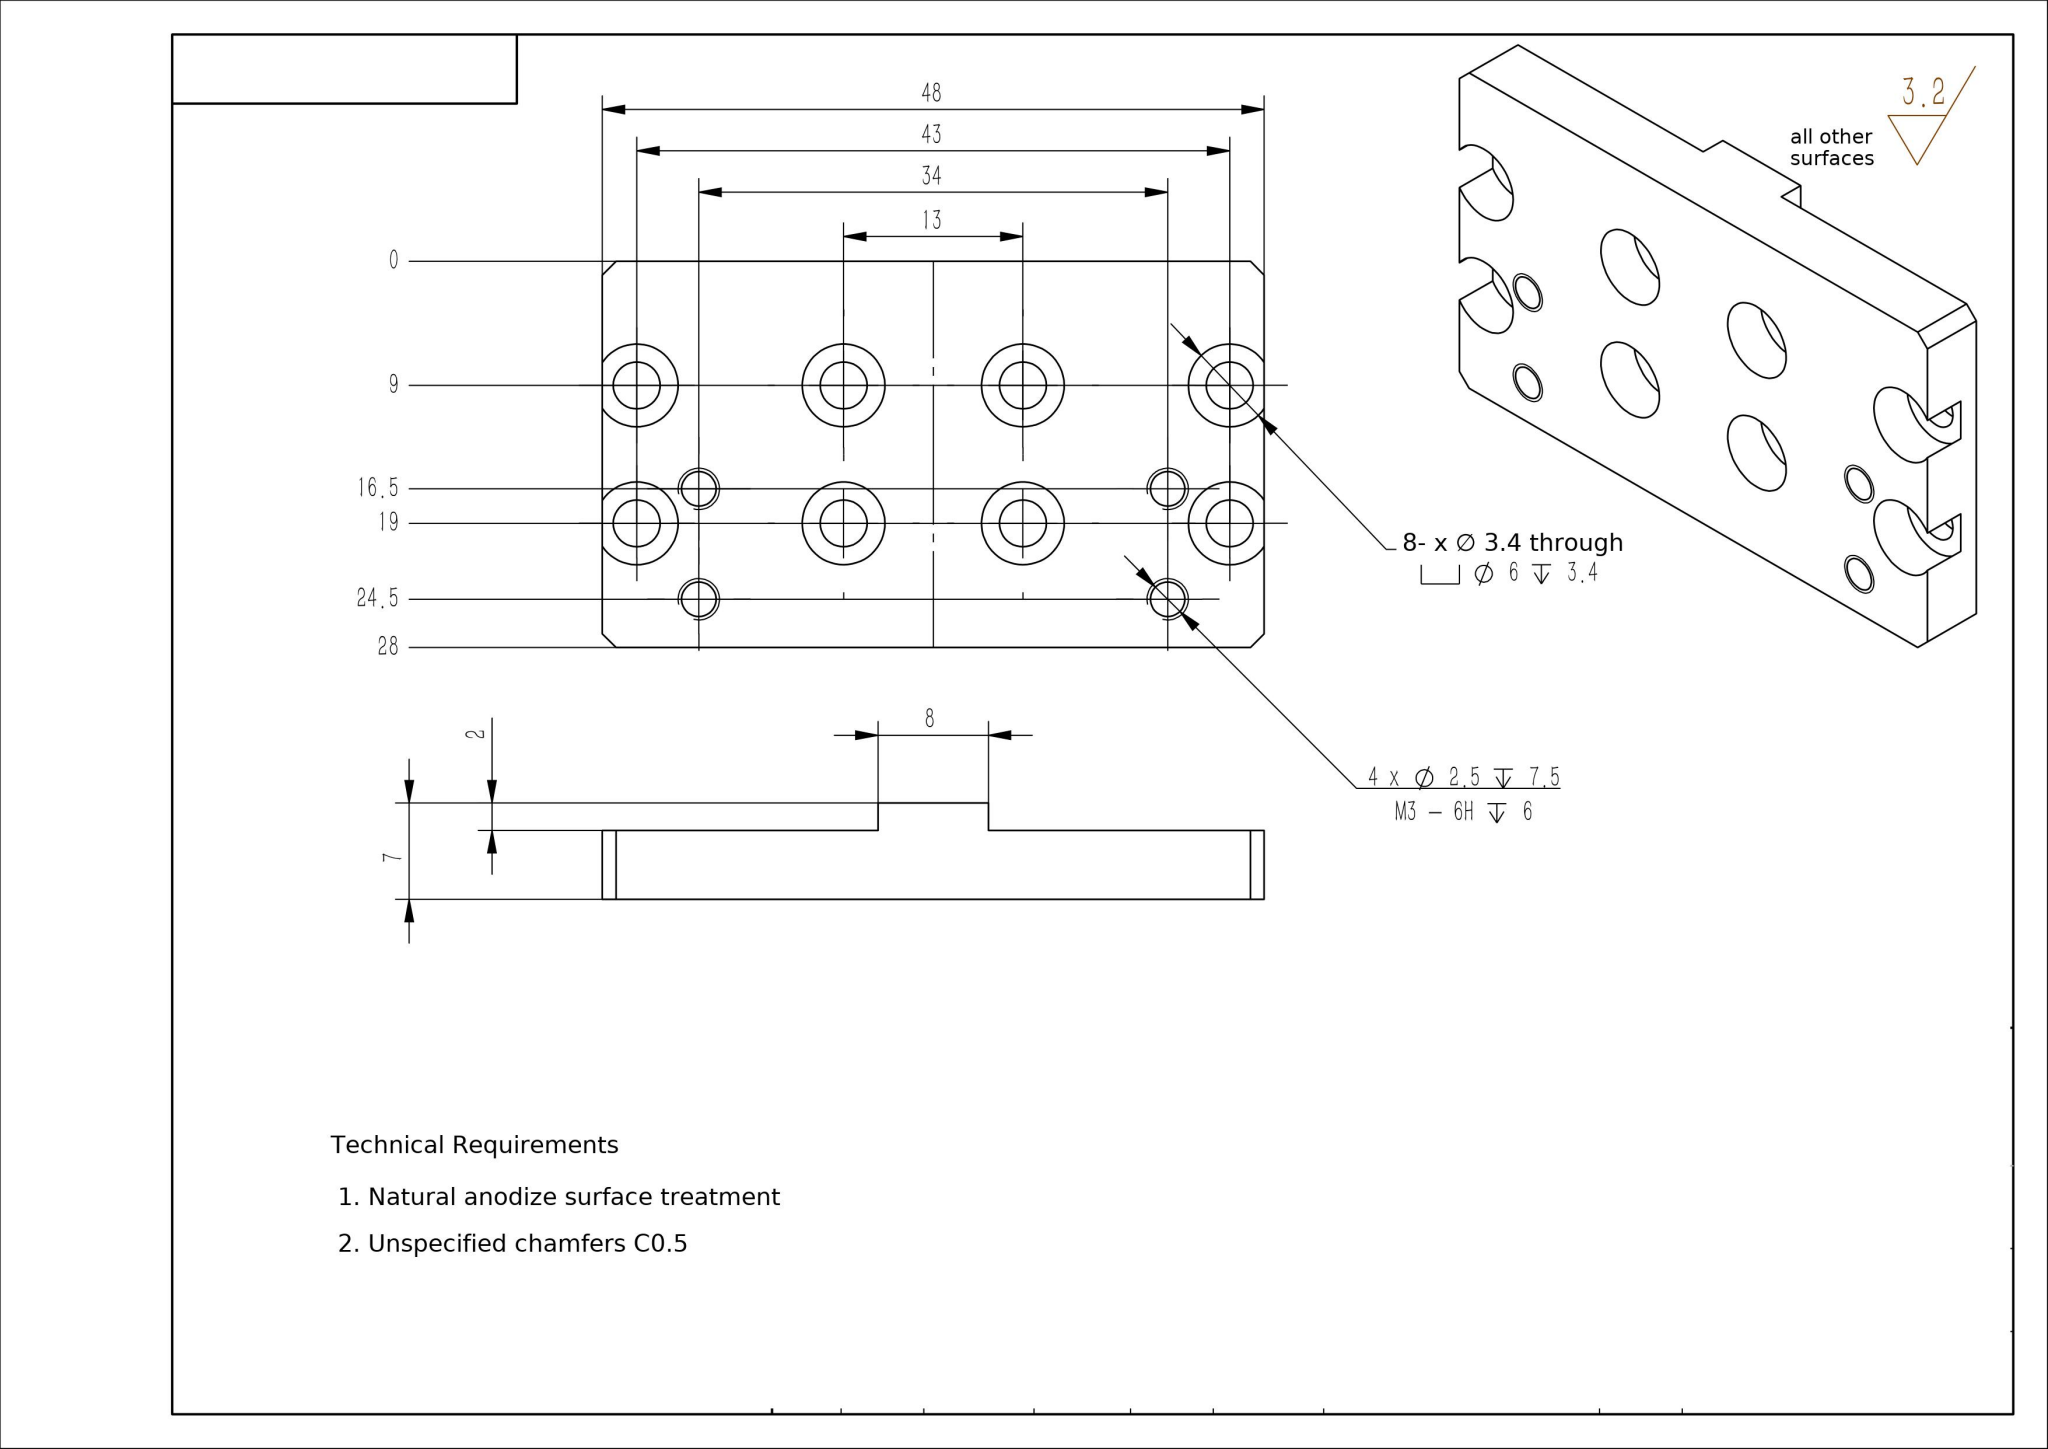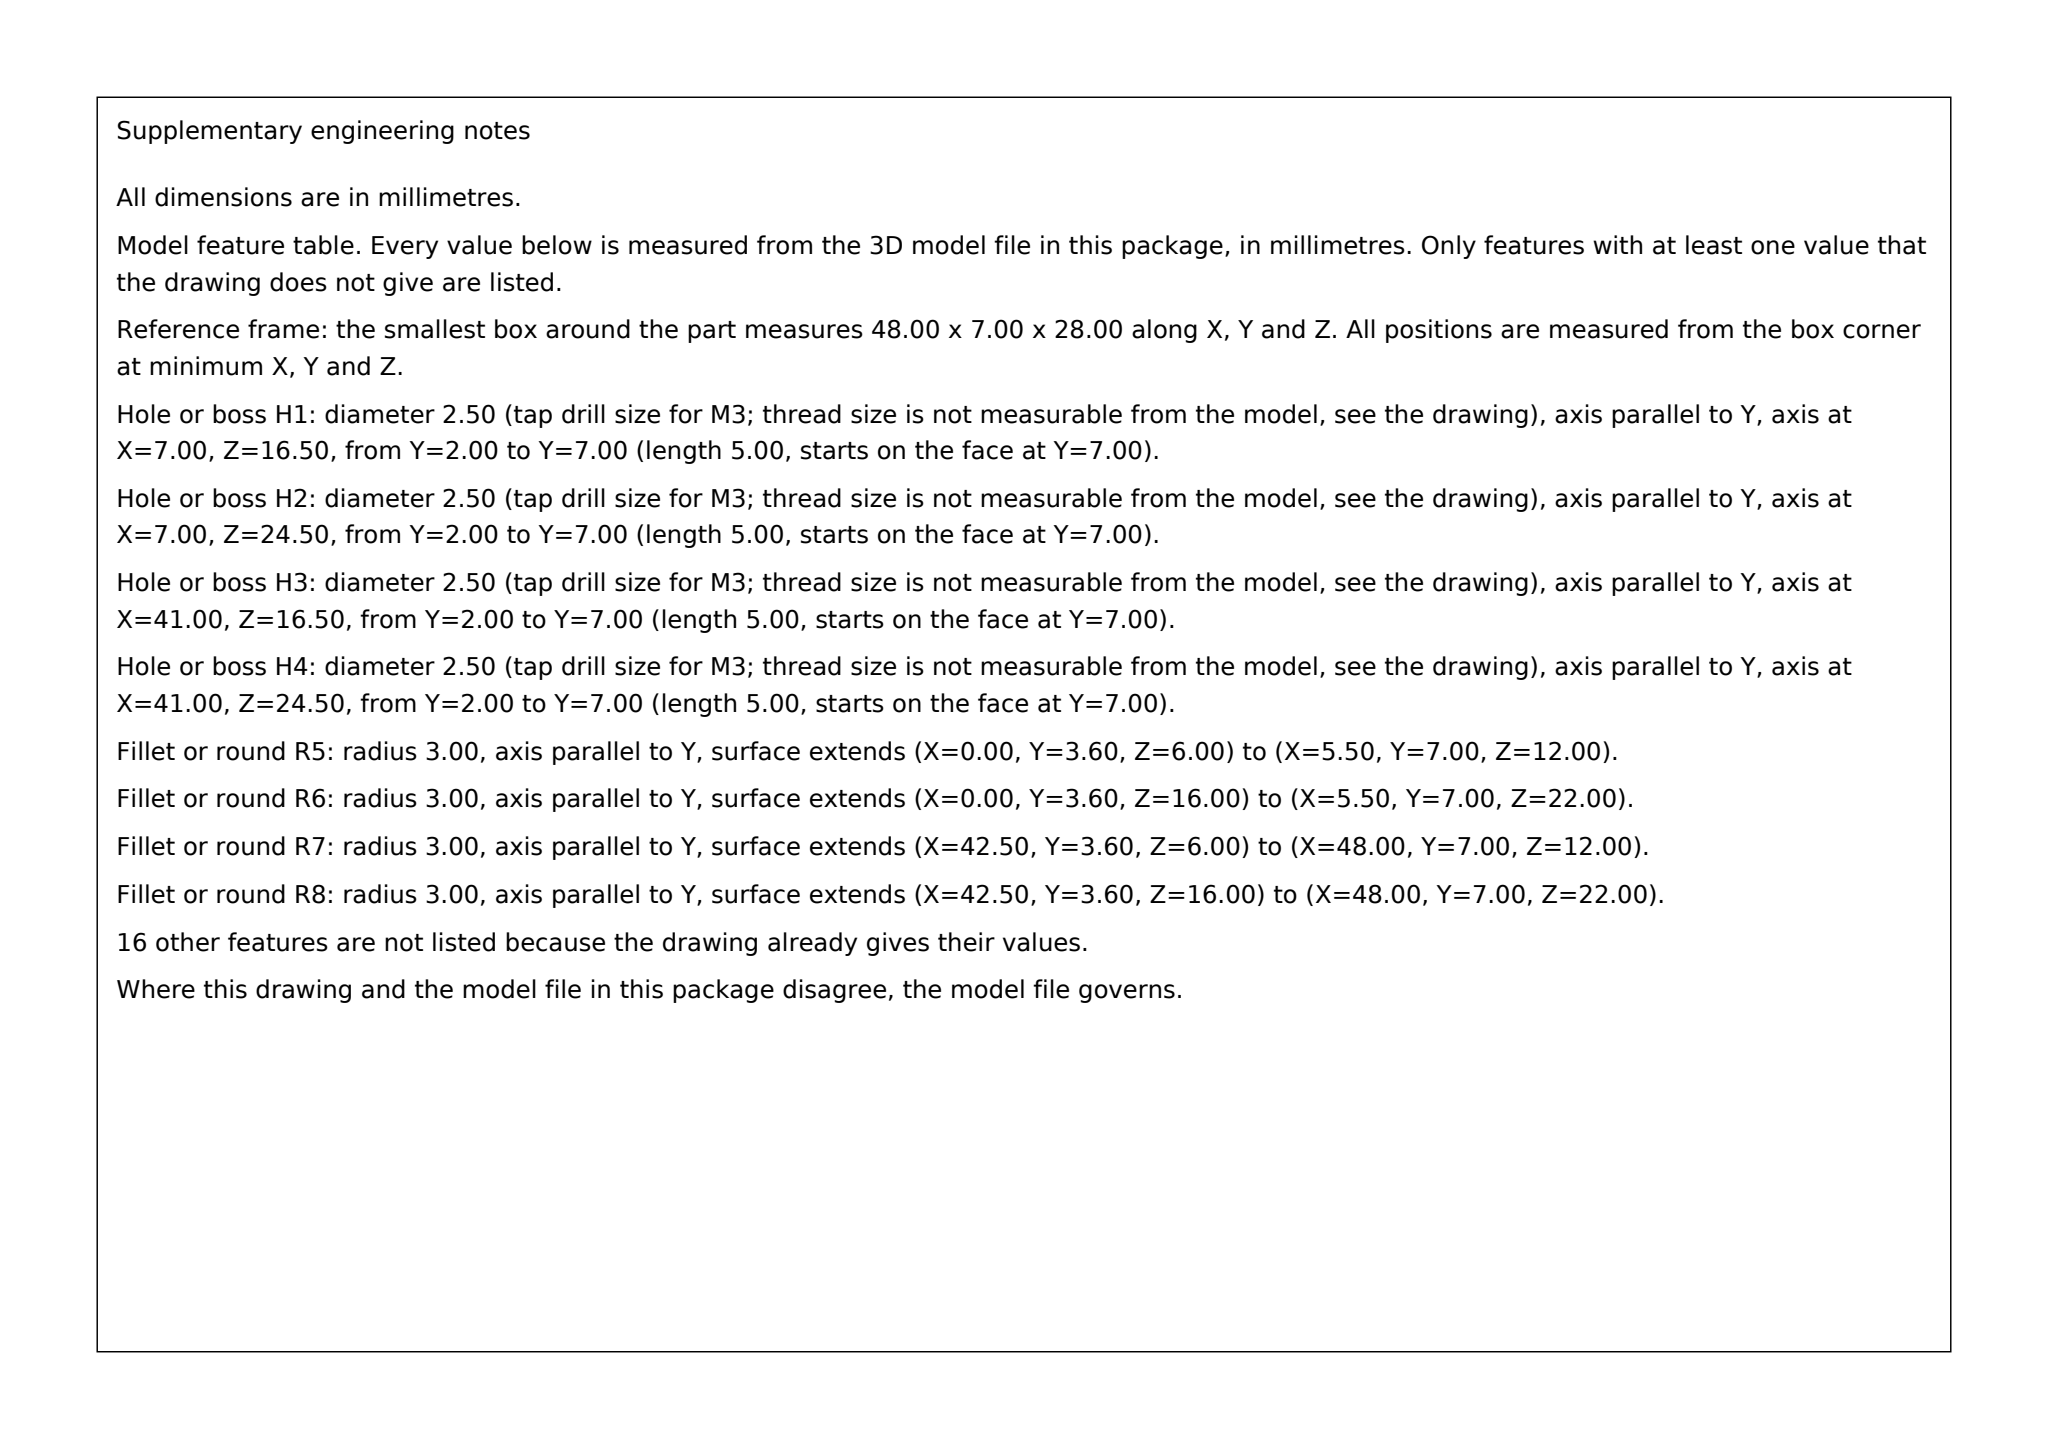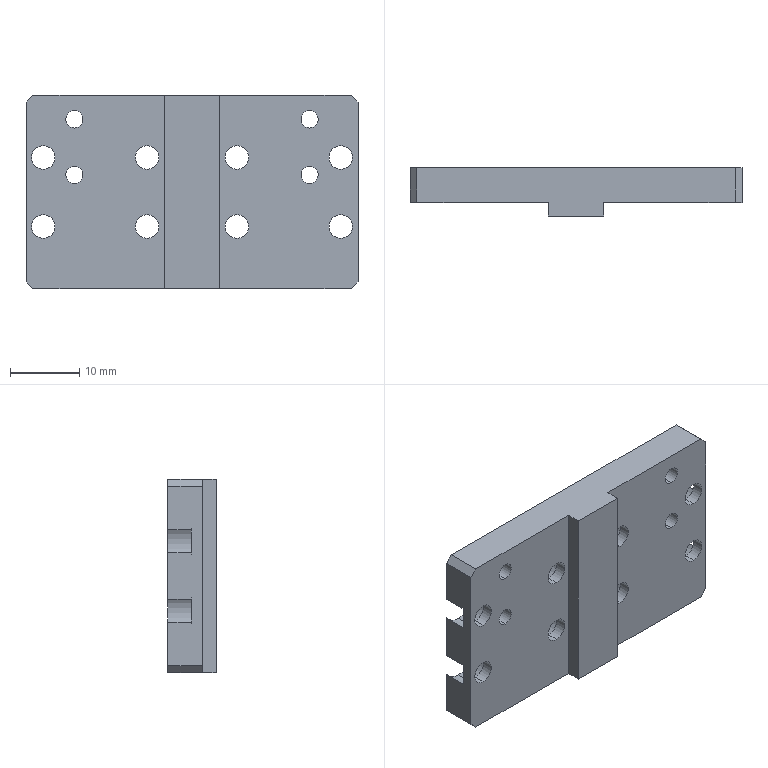Part | SolidWorks | mm | 1 solid | 66 faces | box 48 x 7 x 28 mm | volume 6190 mm3 | cylinder 44 | plane 22 | commonest cylinder face diameters 6 x20 3.4 x16 2.5 x8
build123d program:
from build123d import *

# Parameters (mm, degrees)
SKETCH1_W                                         = 48
SKETCH1_H                                         = 28
BOSS_EXTRUDE1_DEPTH                               = 7
SKETCH4_W                                         = 20
SKETCH4_H                                         = 28
CUT_EXTRUDE2_DEPTH                                = 2
CHAMFER1_SIZE                                     = 1
M3_TAPPED_HOLE2_AT_2_COUNT                        = 2
M3_TAPPED_HOLE2_AT_2_PITCH                        = 8
HOLE_SIZE_ACCORDING_TO_HEXAGON_SOCKET_D           = 3.4
HOLE_SIZE_ACCORDING_TO_HEXAGON_SOCKET_CBORE_D     = 6
HOLE_SIZE_ACCORDING_TO_HEXAGON_SOCKET_CBORE_DEPTH = 3.4


with BuildPart() as part:
    # Sketch1 → Boss-Extrude1 (new body)
    with BuildSketch(Plane(origin=(0, 0, 0), x_dir=(1, 0, 0), z_dir=(0, 1, 0))):
        Rectangle(SKETCH1_W, SKETCH1_H)
    extrude(amount=BOSS_EXTRUDE1_DEPTH)

    # Sketch4 → Cut-Extrude2 (cut)
    with BuildSketch(Plane.XZ):
        with Locations((-14, 0)):
            Rectangle(SKETCH4_W, SKETCH4_H)
        with Locations((14, 0)):
            Rectangle(SKETCH4_W, SKETCH4_H)
    extrude(amount=-CUT_EXTRUDE2_DEPTH, mode=Mode.SUBTRACT)

    # Chamfer1
    chamfer1_edges = [part.edges().sort_by_distance(p)[0] for p in [
        (-24, 4.5, 14),
        (24, 4.5, 14),
        (24, 4.5, -14),
        (-24, 4.5, -14),
    ]]
    chamfer(chamfer1_edges, length=CHAMFER1_SIZE)

    # Sketch9 → M3 Tapped Hole2 (revolve, cut)
    with BuildSketch(Plane(origin=(-17, 7, 2.5), x_dir=(0, 0, 1), z_dir=(1, 0, 0))):
        Polygon((0, 0), (0, 8.251), (1.25, 7.5), (1.25, 0), align=None)
    m3_tapped_hole2 = revolve(axis=Axis((-17, 13.35, 2.5), (0, -1, 0)), mode=Mode.SUBTRACT)

    # M3 Tapped Hole2 at 2: M3 Tapped Hole2 ×2
    with Locations(*[(0, 0, i * M3_TAPPED_HOLE2_AT_2_PITCH) for i in range(1, M3_TAPPED_HOLE2_AT_2_COUNT)]):
        add(m3_tapped_hole2, mode=Mode.SUBTRACT)

    # Hole Size _ according to_ Hexagon Socket (through all)
    with Locations(Plane(origin=(0, 7, 0), x_dir=(1, 0, 0), z_dir=(0, 1, 0))):
        with Locations((-21.5, 5), (-6.5, 5), (-21.5, -5), (-6.5, -5)):
            hole_size_according_to_hexagon_socket = CounterBoreHole(HOLE_SIZE_ACCORDING_TO_HEXAGON_SOCKET_D / 2, HOLE_SIZE_ACCORDING_TO_HEXAGON_SOCKET_CBORE_D / 2, HOLE_SIZE_ACCORDING_TO_HEXAGON_SOCKET_CBORE_DEPTH)

    # Mirror2: M3 Tapped Hole2, Hole Size _ according to_ Hexagon Socket across plane
    add(m3_tapped_hole2.mirror(Plane(origin=(0, 0, 0), x_dir=(0, 0, 1), z_dir=(1, 0, 0))), mode=Mode.SUBTRACT)
    add(hole_size_according_to_hexagon_socket.mirror(Plane(origin=(0, 0, 0), x_dir=(0, 0, 1), z_dir=(1, 0, 0))), mode=Mode.SUBTRACT)

    # Mirror2 copy 1 sketch → Mirror2 copy 1 (revolve, cut)
    with BuildSketch(Plane(origin=(17, 7, 10.5), x_dir=(0, 0, 1), z_dir=(-1, 0, 0))):
        Polygon((0, 0), (0, -8.251), (1.25, -7.5), (1.25, 0), align=None)
    revolve(axis=Axis((17, 13.35, 10.5), (0, 1, 0)), mode=Mode.SUBTRACT)


solid = part.part